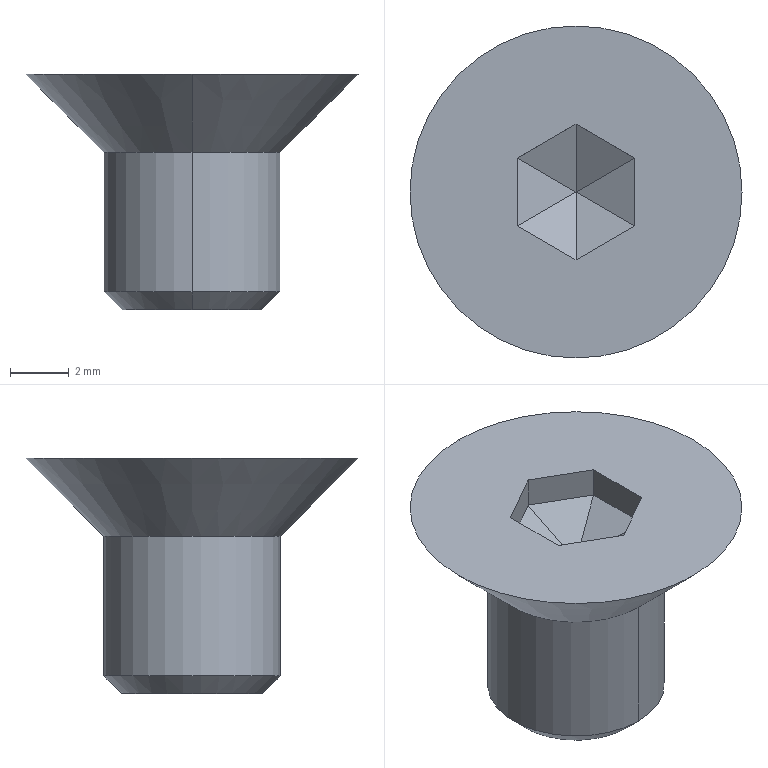Component | SolidWorks | SocketCountersunkHeadScrewM6x8-1 | 1 solid | 21 faces | box 11.3 x 11.3 x 8 mm | volume 289 mm3 | plane 15 | cone 4 | cylinder 2 | commonest cylinder face diameters 6 x2
build123d program:
from build123d import *
from OCP.BRepFilletAPI import BRepFilletAPI_MakeChamfer

# Parameters (mm, degrees)
SKETCH4_R           = 3
BOSS_EXTRUDE2_DEPTH = 8
CUT_EXTRUDE1_DEPTH  = 2.2
CHAMFER3_SIZE       = 1.153
CHAMFER3_SIZE2      = 1.997
CHAMFER4_SIZE       = 0.6


with BuildPart() as part:
    # Sketch2 → Revolve1 (revolve)
    with BuildSketch(Plane.XY, mode=Mode.PRIVATE) as revolve1_sk:
        Polygon((0, -3.72), (0, 0), (5.65, 0), (1.93, -3.72), align=None)
    revolve(revolve1_sk.sketch.rotate(Axis((0, -3.72, 0), (0, 1, 0)), 90), axis=Axis((0, -3.72, 0), (0, 1, 0)))

    # Sketch4 → Boss-Extrude2 (add)
    with BuildSketch(Plane.XZ):
        with Locations(Location((0, 0, 0), (0, 0, 90))):
            Circle(SKETCH4_R)
    extrude(amount=BOSS_EXTRUDE2_DEPTH)

    # Sketch3 → Cut-Extrude1 (cut)
    with BuildSketch(Plane(origin=(0, 0, 0), x_dir=(1, 0, 0), z_dir=(0, 1, 0))):
        Polygon((2, 1.155), (0, 2.309), (-2, 1.155), (-2, -1.155), (0, -2.309), (2, -1.155), align=None)
    extrude(amount=-CUT_EXTRUDE1_DEPTH, mode=Mode.SUBTRACT)

    # Chamfer3: one chamfer whose edges measure the first distance from different faces: ONE call of the kernel's chamfer builder (chamfer() names one face for all edges)
    chamfer3_edges_1 = [part.edges().sort_by_distance(p)[0] for p in [
        (2, -2.2, 0),
    ]]
    chamfer3_side_1 = [part.faces().sort_by_distance(p)[0] for p in [
        (2, -1.1, 0),
    ]]
    chamfer3_edges_2 = [part.edges().sort_by_distance(p)[0] for p in [
        (1, -2.2, 1.732),
    ]]
    chamfer3_side_2 = [part.faces().sort_by_distance(p)[0] for p in [
        (1, -1.1, 1.732),
    ]]
    chamfer3_edges_3 = [part.edges().sort_by_distance(p)[0] for p in [
        (-1, -2.2, 1.732),
    ]]
    chamfer3_side_3 = [part.faces().sort_by_distance(p)[0] for p in [
        (-1, -1.1, 1.732),
    ]]
    chamfer3_edges_4 = [part.edges().sort_by_distance(p)[0] for p in [
        (-2, -2.2, 0),
    ]]
    chamfer3_side_4 = [part.faces().sort_by_distance(p)[0] for p in [
        (-2, -1.1, 0),
    ]]
    chamfer3_edges_5 = [part.edges().sort_by_distance(p)[0] for p in [
        (-1, -2.2, -1.732),
    ]]
    chamfer3_side_5 = [part.faces().sort_by_distance(p)[0] for p in [
        (-1, -1.1, -1.732),
    ]]
    chamfer3_edges_6 = [part.edges().sort_by_distance(p)[0] for p in [
        (1, -2.2, -1.732),
    ]]
    chamfer3_side_6 = [part.faces().sort_by_distance(p)[0] for p in [
        (1, -1.1, -1.732),
    ]]
    chamfer3 = BRepFilletAPI_MakeChamfer(part.part.solid().wrapped)
    for e in chamfer3_edges_1:
        chamfer3.Add(CHAMFER3_SIZE, CHAMFER3_SIZE2, e.wrapped, chamfer3_side_1[0].wrapped)  # the first distance lies on this face
    for e in chamfer3_edges_2:
        chamfer3.Add(CHAMFER3_SIZE, CHAMFER3_SIZE2, e.wrapped, chamfer3_side_2[0].wrapped)  # the first distance lies on this face
    for e in chamfer3_edges_3:
        chamfer3.Add(CHAMFER3_SIZE, CHAMFER3_SIZE2, e.wrapped, chamfer3_side_3[0].wrapped)  # the first distance lies on this face
    for e in chamfer3_edges_4:
        chamfer3.Add(CHAMFER3_SIZE, CHAMFER3_SIZE2, e.wrapped, chamfer3_side_4[0].wrapped)  # the first distance lies on this face
    for e in chamfer3_edges_5:
        chamfer3.Add(CHAMFER3_SIZE, CHAMFER3_SIZE2, e.wrapped, chamfer3_side_5[0].wrapped)  # the first distance lies on this face
    for e in chamfer3_edges_6:
        chamfer3.Add(CHAMFER3_SIZE, CHAMFER3_SIZE2, e.wrapped, chamfer3_side_6[0].wrapped)  # the first distance lies on this face
    add(Compound.cast(chamfer3.Shape()), mode=Mode.REPLACE)

    # Chamfer4
    chamfer4_edges = [part.edges().sort_by_distance(p)[0] for p in [
        (0, -8, -3),
    ]]
    chamfer(chamfer4_edges, length=CHAMFER4_SIZE)


solid = part.part

# Placed as in the assembly
solid = solid.moved(Location((-174.718, -10, 15), (90, 0, 0)))
STEP:
#1=COLOUR_RGB('',0.7922,0.8196,0.9333);
#2=FILL_AREA_STYLE_COLOUR('',#1);
#3=FILL_AREA_STYLE('',(#2));
#4=SURFACE_STYLE_FILL_AREA(#3);
#5=SURFACE_SIDE_STYLE('',(#4));
#6=SURFACE_STYLE_USAGE(.BOTH.,#5);
#7=PRESENTATION_STYLE_ASSIGNMENT((#6));
#8=CARTESIAN_POINT('',(-6.879,-0.2992,0.2756));
#9=VERTEX_POINT('',#8);
#10=CARTESIAN_POINT('',(-6.879,-0.4882,0.2756));
#11=VERTEX_POINT('',#10);
#12=CARTESIAN_POINT('',(-6.879,-0.3937,0.2756));
#13=DIRECTION('',(0.,0.,-1.));
#14=DIRECTION('',(0.,1.,0.));
#15=AXIS2_PLACEMENT_3D('',#12,#13,#14);
#16=CIRCLE('',#15,0.09449);
#17=EDGE_CURVE('',#9,#11,#16,.T.);
#18=ORIENTED_EDGE('',*,*,#17,.F.);
#19=CARTESIAN_POINT('',(-6.879,-0.2756,0.2992));
#20=VERTEX_POINT('',#19);
#21=CARTESIAN_POINT('',(-6.879,-0.2992,0.2756));
#22=DIRECTION('',(0.,0.7071,0.7071));
#23=VECTOR('',#22,39.37);
#24=LINE('',#21,#23);
#25=EDGE_CURVE('',#9,#20,#24,.T.);
#26=ORIENTED_EDGE('',*,*,#25,.T.);
#27=CARTESIAN_POINT('',(-6.879,-0.5118,0.2992));
#28=VERTEX_POINT('',#27);
#29=CARTESIAN_POINT('',(-6.879,-0.3937,0.2992));
#30=DIRECTION('',(0.,-0.,1.));
#31=DIRECTION('',(0.,1.,0.));
#32=AXIS2_PLACEMENT_3D('',#29,#30,#31);
#33=CIRCLE('',#32,0.1181);
#34=EDGE_CURVE('',#28,#20,#33,.T.);
#35=ORIENTED_EDGE('',*,*,#34,.F.);
#36=CARTESIAN_POINT('',(-6.879,-0.4882,0.2756));
#37=DIRECTION('',(0.,-0.7071,0.7071));
#38=VECTOR('',#37,39.37);
#39=LINE('',#36,#38);
#40=EDGE_CURVE('',#11,#28,#39,.T.);
#41=ORIENTED_EDGE('',*,*,#40,.F.);
#42=EDGE_LOOP('',(#18,#26,#35,#41));
#43=FACE_OUTER_BOUND('',#42,.T.);
#44=CARTESIAN_POINT('',(-6.879,-0.3937,0.2756));
#45=DIRECTION('',(0.,-0.,1.));
#46=DIRECTION('',(0.,-1.,-0.));
#47=AXIS2_PLACEMENT_3D('',#44,#45,#46);
#48=CONICAL_SURFACE('',#47,0.09449,0.7854);
#49=ADVANCED_FACE('',(#43),#48,.T.);
#50=ORIENTED_EDGE('',*,*,#34,.T.);
#51=CARTESIAN_POINT('',(-6.879,-0.2756,0.4862));
#52=VERTEX_POINT('',#51);
#53=CARTESIAN_POINT('',(-6.879,-0.2756,0.2756));
#54=DIRECTION('',(0.,-0.,1.));
#55=VECTOR('',#54,39.37);
#56=LINE('',#53,#55);
#57=EDGE_CURVE('',#20,#52,#56,.T.);
#58=ORIENTED_EDGE('',*,*,#57,.T.);
#59=CARTESIAN_POINT('',(-6.879,-0.5118,0.4862));
#60=VERTEX_POINT('',#59);
#61=CARTESIAN_POINT('',(-6.879,-0.3937,0.4862));
#62=DIRECTION('',(0.,-0.,1.));
#63=DIRECTION('',(0.,-1.,-0.));
#64=AXIS2_PLACEMENT_3D('',#61,#62,#63);
#65=CIRCLE('',#64,0.1181);
#66=EDGE_CURVE('',#60,#52,#65,.T.);
#67=ORIENTED_EDGE('',*,*,#66,.F.);
#68=CARTESIAN_POINT('',(-6.879,-0.5118,0.2756));
#69=DIRECTION('',(0.,-0.,1.));
#70=VECTOR('',#69,39.37);
#71=LINE('',#68,#70);
#72=EDGE_CURVE('',#28,#60,#71,.T.);
#73=ORIENTED_EDGE('',*,*,#72,.F.);
#74=EDGE_LOOP('',(#50,#58,#67,#73));
#75=FACE_OUTER_BOUND('',#74,.T.);
#76=CARTESIAN_POINT('',(-6.879,-0.3937,0.2756));
#77=DIRECTION('',(0.,-0.,1.));
#78=DIRECTION('',(0.,-1.,-0.));
#79=AXIS2_PLACEMENT_3D('',#76,#77,#78);
#80=CYLINDRICAL_SURFACE('',#79,0.1181);
#81=ADVANCED_FACE('',(#75),#80,.T.);
#82=ORIENTED_EDGE('',*,*,#66,.T.);
#83=CARTESIAN_POINT('',(-6.879,-0.1713,0.5906));
#84=VERTEX_POINT('',#83);
#85=CARTESIAN_POINT('',(-6.879,-0.3177,0.4441));
#86=DIRECTION('',(0.,0.7071,0.7071));
#87=VECTOR('',#86,39.37);
#88=LINE('',#85,#87);
#89=EDGE_CURVE('',#52,#84,#88,.T.);
#90=ORIENTED_EDGE('',*,*,#89,.T.);
#91=CARTESIAN_POINT('',(-6.879,-0.6161,0.5906));
#92=VERTEX_POINT('',#91);
#93=CARTESIAN_POINT('',(-6.879,-0.3937,0.5906));
#94=DIRECTION('',(0.,0.,-1.));
#95=DIRECTION('',(0.,1.,0.));
#96=AXIS2_PLACEMENT_3D('',#93,#94,#95);
#97=CIRCLE('',#96,0.2224);
#98=EDGE_CURVE('',#84,#92,#97,.T.);
#99=ORIENTED_EDGE('',*,*,#98,.T.);
#100=CARTESIAN_POINT('',(-6.879,-0.4697,0.4441));
#101=DIRECTION('',(0.,-0.7071,0.7071));
#102=VECTOR('',#101,39.37);
#103=LINE('',#100,#102);
#104=EDGE_CURVE('',#60,#92,#103,.T.);
#105=ORIENTED_EDGE('',*,*,#104,.F.);
#106=EDGE_LOOP('',(#82,#90,#99,#105));
#107=FACE_OUTER_BOUND('',#106,.T.);
#108=CARTESIAN_POINT('',(-6.879,-0.3937,0.4441));
#109=DIRECTION('',(0.,-0.,1.));
#110=DIRECTION('',(0.,-1.,-0.));
#111=AXIS2_PLACEMENT_3D('',#108,#109,#110);
#112=CONICAL_SURFACE('',#111,0.07598,0.7854);
#113=ADVANCED_FACE('',(#107),#112,.T.);
#114=ORIENTED_EDGE('',*,*,#89,.F.);
#115=CARTESIAN_POINT('',(-6.879,-0.3937,0.4862));
#116=DIRECTION('',(0.,-0.,1.));
#117=DIRECTION('',(0.,-1.,-0.));
#118=AXIS2_PLACEMENT_3D('',#115,#116,#117);
#119=CIRCLE('',#118,0.1181);
#120=EDGE_CURVE('',#52,#60,#119,.T.);
#121=ORIENTED_EDGE('',*,*,#120,.T.);
#122=ORIENTED_EDGE('',*,*,#104,.T.);
#123=CARTESIAN_POINT('',(-6.879,-0.3937,0.5906));
#124=DIRECTION('',(0.,0.,-1.));
#125=DIRECTION('',(0.,1.,0.));
#126=AXIS2_PLACEMENT_3D('',#123,#124,#125);
#127=CIRCLE('',#126,0.2224);
#128=EDGE_CURVE('',#92,#84,#127,.T.);
#129=ORIENTED_EDGE('',*,*,#128,.T.);
#130=EDGE_LOOP('',(#114,#121,#122,#129));
#131=FACE_OUTER_BOUND('',#130,.T.);
#132=CARTESIAN_POINT('',(-6.879,-0.3937,0.4441));
#133=DIRECTION('',(0.,-0.,1.));
#134=DIRECTION('',(0.,-1.,-0.));
#135=AXIS2_PLACEMENT_3D('',#132,#133,#134);
#136=CONICAL_SURFACE('',#135,0.07598,0.7854);
#137=ADVANCED_FACE('',(#131),#136,.T.);
#138=CARTESIAN_POINT('',(-6.8,-0.4392,0.5906));
#139=VERTEX_POINT('',#138);
#140=CARTESIAN_POINT('',(-6.8,-0.3482,0.5906));
#141=VERTEX_POINT('',#140);
#142=CARTESIAN_POINT('',(-6.8,-0.4392,0.5906));
#143=DIRECTION('',(-0.,1.,0.));
#144=VECTOR('',#143,39.37);
#145=LINE('',#142,#144);
#146=EDGE_CURVE('',#139,#141,#145,.T.);
#147=ORIENTED_EDGE('',*,*,#146,.F.);
#148=CARTESIAN_POINT('',(-6.879,-0.4846,0.5906));
#149=VERTEX_POINT('',#148);
#150=CARTESIAN_POINT('',(-6.879,-0.4846,0.5906));
#151=DIRECTION('',(0.866,0.5,0.));
#152=VECTOR('',#151,39.37);
#153=LINE('',#150,#152);
#154=EDGE_CURVE('',#149,#139,#153,.T.);
#155=ORIENTED_EDGE('',*,*,#154,.F.);
#156=CARTESIAN_POINT('',(-6.957,-0.4392,0.5906));
#157=VERTEX_POINT('',#156);
#158=CARTESIAN_POINT('',(-6.957,-0.4392,0.5906));
#159=DIRECTION('',(0.866,-0.5,-0.));
#160=VECTOR('',#159,39.37);
#161=LINE('',#158,#160);
#162=EDGE_CURVE('',#157,#149,#161,.T.);
#163=ORIENTED_EDGE('',*,*,#162,.F.);
#164=CARTESIAN_POINT('',(-6.957,-0.3482,0.5906));
#165=VERTEX_POINT('',#164);
#166=CARTESIAN_POINT('',(-6.957,-0.3482,0.5906));
#167=DIRECTION('',(0.,-1.,-0.));
#168=VECTOR('',#167,39.37);
#169=LINE('',#166,#168);
#170=EDGE_CURVE('',#165,#157,#169,.T.);
#171=ORIENTED_EDGE('',*,*,#170,.F.);
#172=CARTESIAN_POINT('',(-6.879,-0.3028,0.5906));
#173=VERTEX_POINT('',#172);
#174=CARTESIAN_POINT('',(-6.879,-0.3028,0.5906));
#175=DIRECTION('',(-0.866,-0.5,-0.));
#176=VECTOR('',#175,39.37);
#177=LINE('',#174,#176);
#178=EDGE_CURVE('',#173,#165,#177,.T.);
#179=ORIENTED_EDGE('',*,*,#178,.F.);
#180=CARTESIAN_POINT('',(-6.8,-0.3482,0.5906));
#181=DIRECTION('',(-0.866,0.5,0.));
#182=VECTOR('',#181,39.37);
#183=LINE('',#180,#182);
#184=EDGE_CURVE('',#141,#173,#183,.T.);
#185=ORIENTED_EDGE('',*,*,#184,.F.);
#186=EDGE_LOOP('',(#147,#155,#163,#171,#179,#185));
#187=FACE_BOUND('',#186,.T.);
#188=ORIENTED_EDGE('',*,*,#128,.F.);
#189=ORIENTED_EDGE('',*,*,#98,.F.);
#190=EDGE_LOOP('',(#188,#189));
#191=FACE_OUTER_BOUND('',#190,.T.);
#192=CARTESIAN_POINT('',(-6.879,-0.3937,0.5906));
#193=DIRECTION('',(0.,-0.,1.));
#194=DIRECTION('',(0.,-1.,-0.));
#195=AXIS2_PLACEMENT_3D('',#192,#193,#194);
#196=PLANE('',#195);
#197=ADVANCED_FACE('',(#187,#191),#196,.T.);
#198=ORIENTED_EDGE('',*,*,#57,.F.);
#199=CARTESIAN_POINT('',(-6.879,-0.3937,0.2992));
#200=DIRECTION('',(0.,-0.,1.));
#201=DIRECTION('',(0.,1.,0.));
#202=AXIS2_PLACEMENT_3D('',#199,#200,#201);
#203=CIRCLE('',#202,0.1181);
#204=EDGE_CURVE('',#20,#28,#203,.T.);
#205=ORIENTED_EDGE('',*,*,#204,.T.);
#206=ORIENTED_EDGE('',*,*,#72,.T.);
#207=ORIENTED_EDGE('',*,*,#120,.F.);
#208=EDGE_LOOP('',(#198,#205,#206,#207));
#209=FACE_OUTER_BOUND('',#208,.T.);
#210=CARTESIAN_POINT('',(-6.879,-0.3937,0.2756));
#211=DIRECTION('',(0.,-0.,1.));
#212=DIRECTION('',(0.,-1.,-0.));
#213=AXIS2_PLACEMENT_3D('',#210,#211,#212);
#214=CYLINDRICAL_SURFACE('',#213,0.1181);
#215=ADVANCED_FACE('',(#209),#214,.T.);
#216=CARTESIAN_POINT('',(-6.879,-0.3937,0.2756));
#217=DIRECTION('',(0.,0.,-1.));
#218=DIRECTION('',(0.,1.,0.));
#219=AXIS2_PLACEMENT_3D('',#216,#217,#218);
#220=CIRCLE('',#219,0.09449);
#221=EDGE_CURVE('',#11,#9,#220,.T.);
#222=ORIENTED_EDGE('',*,*,#221,.T.);
#223=ORIENTED_EDGE('',*,*,#17,.T.);
#224=EDGE_LOOP('',(#222,#223));
#225=FACE_OUTER_BOUND('',#224,.T.);
#226=CARTESIAN_POINT('',(-6.879,-0.3937,0.2756));
#227=DIRECTION('',(0.,0.,-1.));
#228=DIRECTION('',(0.,1.,0.));
#229=AXIS2_PLACEMENT_3D('',#226,#227,#228);
#230=PLANE('',#229);
#231=ADVANCED_FACE('',(#225),#230,.T.);
#232=CARTESIAN_POINT('',(-6.8,-0.3482,0.5493));
#233=VERTEX_POINT('',#232);
#234=CARTESIAN_POINT('',(-6.8,-0.3482,0.5039));
#235=DIRECTION('',(0.,-0.,1.));
#236=VECTOR('',#235,39.37);
#237=LINE('',#234,#236);
#238=EDGE_CURVE('',#233,#141,#237,.T.);
#239=ORIENTED_EDGE('',*,*,#238,.F.);
#240=CARTESIAN_POINT('',(-6.8,-0.4392,0.5493));
#241=VERTEX_POINT('',#240);
#242=CARTESIAN_POINT('',(-6.8,-0.4392,0.5493));
#243=DIRECTION('',(0.,-1.,-0.));
#244=VECTOR('',#243,39.37);
#245=LINE('',#242,#244);
#246=EDGE_CURVE('',#233,#241,#245,.T.);
#247=ORIENTED_EDGE('',*,*,#246,.T.);
#248=CARTESIAN_POINT('',(-6.8,-0.4392,0.5039));
#249=DIRECTION('',(0.,-0.,1.));
#250=VECTOR('',#249,39.37);
#251=LINE('',#248,#250);
#252=EDGE_CURVE('',#241,#139,#251,.T.);
#253=ORIENTED_EDGE('',*,*,#252,.T.);
#254=ORIENTED_EDGE('',*,*,#146,.T.);
#255=EDGE_LOOP('',(#239,#247,#253,#254));
#256=FACE_OUTER_BOUND('',#255,.T.);
#257=CARTESIAN_POINT('',(-6.8,-0.4392,0.5039));
#258=DIRECTION('',(1.,0.,0.));
#259=DIRECTION('',(-0.,1.,0.));
#260=AXIS2_PLACEMENT_3D('',#257,#258,#259);
#261=PLANE('',#260);
#262=ADVANCED_FACE('',(#256),#261,.F.);
#263=ORIENTED_EDGE('',*,*,#252,.F.);
#264=CARTESIAN_POINT('',(-6.879,-0.4846,0.5493));
#265=VERTEX_POINT('',#264);
#266=CARTESIAN_POINT('',(-6.879,-0.4846,0.5493));
#267=DIRECTION('',(-0.866,-0.5,-0.));
#268=VECTOR('',#267,39.37);
#269=LINE('',#266,#268);
#270=EDGE_CURVE('',#241,#265,#269,.T.);
#271=ORIENTED_EDGE('',*,*,#270,.T.);
#272=CARTESIAN_POINT('',(-6.879,-0.4846,0.5039));
#273=DIRECTION('',(0.,-0.,1.));
#274=VECTOR('',#273,39.37);
#275=LINE('',#272,#274);
#276=EDGE_CURVE('',#265,#149,#275,.T.);
#277=ORIENTED_EDGE('',*,*,#276,.T.);
#278=ORIENTED_EDGE('',*,*,#154,.T.);
#279=EDGE_LOOP('',(#263,#271,#277,#278));
#280=FACE_OUTER_BOUND('',#279,.T.);
#281=CARTESIAN_POINT('',(-6.879,-0.4846,0.5039));
#282=DIRECTION('',(0.5,-0.866,-0.));
#283=DIRECTION('',(0.866,0.5,0.));
#284=AXIS2_PLACEMENT_3D('',#281,#282,#283);
#285=PLANE('',#284);
#286=ADVANCED_FACE('',(#280),#285,.F.);
#287=ORIENTED_EDGE('',*,*,#276,.F.);
#288=CARTESIAN_POINT('',(-6.957,-0.4392,0.5493));
#289=VERTEX_POINT('',#288);
#290=CARTESIAN_POINT('',(-6.957,-0.4392,0.5493));
#291=DIRECTION('',(-0.866,0.5,0.));
#292=VECTOR('',#291,39.37);
#293=LINE('',#290,#292);
#294=EDGE_CURVE('',#265,#289,#293,.T.);
#295=ORIENTED_EDGE('',*,*,#294,.T.);
#296=CARTESIAN_POINT('',(-6.957,-0.4392,0.5039));
#297=DIRECTION('',(0.,-0.,1.));
#298=VECTOR('',#297,39.37);
#299=LINE('',#296,#298);
#300=EDGE_CURVE('',#289,#157,#299,.T.);
#301=ORIENTED_EDGE('',*,*,#300,.T.);
#302=ORIENTED_EDGE('',*,*,#162,.T.);
#303=EDGE_LOOP('',(#287,#295,#301,#302));
#304=FACE_OUTER_BOUND('',#303,.T.);
#305=CARTESIAN_POINT('',(-6.957,-0.4392,0.5039));
#306=DIRECTION('',(-0.5,-0.866,-0.));
#307=DIRECTION('',(0.866,-0.5,-0.));
#308=AXIS2_PLACEMENT_3D('',#305,#306,#307);
#309=PLANE('',#308);
#310=ADVANCED_FACE('',(#304),#309,.F.);
#311=ORIENTED_EDGE('',*,*,#300,.F.);
#312=CARTESIAN_POINT('',(-6.957,-0.3482,0.5493));
#313=VERTEX_POINT('',#312);
#314=CARTESIAN_POINT('',(-6.957,-0.3482,0.5493));
#315=DIRECTION('',(0.,1.,0.));
#316=VECTOR('',#315,39.37);
#317=LINE('',#314,#316);
#318=EDGE_CURVE('',#289,#313,#317,.T.);
#319=ORIENTED_EDGE('',*,*,#318,.T.);
#320=CARTESIAN_POINT('',(-6.957,-0.3482,0.5039));
#321=DIRECTION('',(0.,-0.,1.));
#322=VECTOR('',#321,39.37);
#323=LINE('',#320,#322);
#324=EDGE_CURVE('',#313,#165,#323,.T.);
#325=ORIENTED_EDGE('',*,*,#324,.T.);
#326=ORIENTED_EDGE('',*,*,#170,.T.);
#327=EDGE_LOOP('',(#311,#319,#325,#326));
#328=FACE_OUTER_BOUND('',#327,.T.);
#329=CARTESIAN_POINT('',(-6.957,-0.3482,0.5039));
#330=DIRECTION('',(-1.,0.,0.));
#331=DIRECTION('',(0.,-1.,-0.));
#332=AXIS2_PLACEMENT_3D('',#329,#330,#331);
#333=PLANE('',#332);
#334=ADVANCED_FACE('',(#328),#333,.F.);
#335=ORIENTED_EDGE('',*,*,#324,.F.);
#336=CARTESIAN_POINT('',(-6.879,-0.3028,0.5493));
#337=VERTEX_POINT('',#336);
#338=CARTESIAN_POINT('',(-6.879,-0.3028,0.5493));
#339=DIRECTION('',(0.866,0.5,0.));
#340=VECTOR('',#339,39.37);
#341=LINE('',#338,#340);
#342=EDGE_CURVE('',#313,#337,#341,.T.);
#343=ORIENTED_EDGE('',*,*,#342,.T.);
#344=CARTESIAN_POINT('',(-6.879,-0.3028,0.5039));
#345=DIRECTION('',(0.,-0.,1.));
#346=VECTOR('',#345,39.37);
#347=LINE('',#344,#346);
#348=EDGE_CURVE('',#337,#173,#347,.T.);
#349=ORIENTED_EDGE('',*,*,#348,.T.);
#350=ORIENTED_EDGE('',*,*,#178,.T.);
#351=EDGE_LOOP('',(#335,#343,#349,#350));
#352=FACE_OUTER_BOUND('',#351,.T.);
#353=CARTESIAN_POINT('',(-6.879,-0.3028,0.5039));
#354=DIRECTION('',(-0.5,0.866,0.));
#355=DIRECTION('',(-0.866,-0.5,-0.));
#356=AXIS2_PLACEMENT_3D('',#353,#354,#355);
#357=PLANE('',#356);
#358=ADVANCED_FACE('',(#352),#357,.F.);
#359=ORIENTED_EDGE('',*,*,#348,.F.);
#360=CARTESIAN_POINT('',(-6.8,-0.3482,0.5493));
#361=DIRECTION('',(0.866,-0.5,-0.));
#362=VECTOR('',#361,39.37);
#363=LINE('',#360,#362);
#364=EDGE_CURVE('',#337,#233,#363,.T.);
#365=ORIENTED_EDGE('',*,*,#364,.T.);
#366=ORIENTED_EDGE('',*,*,#238,.T.);
#367=ORIENTED_EDGE('',*,*,#184,.T.);
#368=EDGE_LOOP('',(#359,#365,#366,#367));
#369=FACE_OUTER_BOUND('',#368,.T.);
#370=CARTESIAN_POINT('',(-6.8,-0.3482,0.5039));
#371=DIRECTION('',(0.5,0.866,0.));
#372=DIRECTION('',(-0.866,0.5,0.));
#373=AXIS2_PLACEMENT_3D('',#370,#371,#372);
#374=PLANE('',#373);
#375=ADVANCED_FACE('',(#369),#374,.F.);
#376=CARTESIAN_POINT('',(-6.879,-0.3936,0.5039));
#377=VERTEX_POINT('',#376);
#378=CARTESIAN_POINT('',(-6.879,-0.3938,0.5039));
#379=VERTEX_POINT('',#378);
#380=CARTESIAN_POINT('',(-6.879,-0.3937,0.5039));
#381=DIRECTION('',(0.,-1.,-0.));
#382=VECTOR('',#381,39.37);
#383=LINE('',#380,#382);
#384=EDGE_CURVE('',#377,#379,#383,.T.);
#385=ORIENTED_EDGE('',*,*,#384,.T.);
#386=CARTESIAN_POINT('',(-6.879,-0.3939,0.5039));
#387=VERTEX_POINT('',#386);
#388=CARTESIAN_POINT('',(-6.879,-0.3938,0.5039));
#389=DIRECTION('',(0.866,-0.5,-0.));
#390=VECTOR('',#389,39.37);
#391=LINE('',#388,#390);
#392=EDGE_CURVE('',#379,#387,#391,.T.);
#393=ORIENTED_EDGE('',*,*,#392,.T.);
#394=CARTESIAN_POINT('',(-6.879,-0.3938,0.5039));
#395=VERTEX_POINT('',#394);
#396=CARTESIAN_POINT('',(-6.879,-0.3938,0.5039));
#397=DIRECTION('',(0.866,0.5,0.));
#398=VECTOR('',#397,39.37);
#399=LINE('',#396,#398);
#400=EDGE_CURVE('',#387,#395,#399,.T.);
#401=ORIENTED_EDGE('',*,*,#400,.T.);
#402=CARTESIAN_POINT('',(-6.879,-0.3936,0.5039));
#403=VERTEX_POINT('',#402);
#404=CARTESIAN_POINT('',(-6.879,-0.3937,0.5039));
#405=DIRECTION('',(-0.,1.,0.));
#406=VECTOR('',#405,39.37);
#407=LINE('',#404,#406);
#408=EDGE_CURVE('',#395,#403,#407,.T.);
#409=ORIENTED_EDGE('',*,*,#408,.T.);
#410=CARTESIAN_POINT('',(-6.879,-0.3935,0.5039));
#411=VERTEX_POINT('',#410);
#412=CARTESIAN_POINT('',(-6.879,-0.3936,0.5039));
#413=DIRECTION('',(-0.866,0.5,0.));
#414=VECTOR('',#413,39.37);
#415=LINE('',#412,#414);
#416=EDGE_CURVE('',#403,#411,#415,.T.);
#417=ORIENTED_EDGE('',*,*,#416,.T.);
#418=CARTESIAN_POINT('',(-6.879,-0.3936,0.5039));
#419=DIRECTION('',(-0.866,-0.5,-0.));
#420=VECTOR('',#419,39.37);
#421=LINE('',#418,#420);
#422=EDGE_CURVE('',#411,#377,#421,.T.);
#423=ORIENTED_EDGE('',*,*,#422,.T.);
#424=EDGE_LOOP('',(#385,#393,#401,#409,#417,#423));
#425=FACE_OUTER_BOUND('',#424,.T.);
#426=CARTESIAN_POINT('',(-6.879,-0.3937,0.5039));
#427=DIRECTION('',(0.,-0.,1.));
#428=DIRECTION('',(0.,-1.,-0.));
#429=AXIS2_PLACEMENT_3D('',#426,#427,#428);
#430=PLANE('',#429);
#431=ADVANCED_FACE('',(#425),#430,.T.);
#432=CARTESIAN_POINT('',(-6.879,-0.3936,0.5039));
#433=DIRECTION('',(-0.7746,-0.4472,-0.4472));
#434=VECTOR('',#433,39.37);
#435=LINE('',#432,#434);
#436=EDGE_CURVE('',#233,#403,#435,.T.);
#437=ORIENTED_EDGE('',*,*,#436,.F.);
#438=ORIENTED_EDGE('',*,*,#364,.F.);
#439=CARTESIAN_POINT('',(-6.879,-0.3936,0.5039));
#440=DIRECTION('',(0.,0.8944,0.4472));
#441=VECTOR('',#440,39.37);
#442=LINE('',#439,#441);
#443=EDGE_CURVE('',#411,#337,#442,.T.);
#444=ORIENTED_EDGE('',*,*,#443,.F.);
#445=ORIENTED_EDGE('',*,*,#416,.F.);
#446=EDGE_LOOP('',(#437,#438,#444,#445));
#447=FACE_OUTER_BOUND('',#446,.T.);
#448=CARTESIAN_POINT('',(-6.879,-0.3936,0.5039));
#449=DIRECTION('',(0.25,0.433,-0.866));
#450=DIRECTION('',(-0.866,0.5,0.));
#451=AXIS2_PLACEMENT_3D('',#448,#449,#450);
#452=PLANE('',#451);
#453=ADVANCED_FACE('',(#447),#452,.F.);
#454=ORIENTED_EDGE('',*,*,#443,.T.);
#455=ORIENTED_EDGE('',*,*,#342,.F.);
#456=CARTESIAN_POINT('',(-6.879,-0.3936,0.5039));
#457=DIRECTION('',(-0.7746,0.4472,0.4472));
#458=VECTOR('',#457,39.37);
#459=LINE('',#456,#458);
#460=EDGE_CURVE('',#377,#313,#459,.T.);
#461=ORIENTED_EDGE('',*,*,#460,.F.);
#462=ORIENTED_EDGE('',*,*,#422,.F.);
#463=EDGE_LOOP('',(#454,#455,#461,#462));
#464=FACE_OUTER_BOUND('',#463,.T.);
#465=CARTESIAN_POINT('',(-6.879,-0.3936,0.5039));
#466=DIRECTION('',(-0.25,0.433,-0.866));
#467=DIRECTION('',(-0.866,-0.5,-0.));
#468=AXIS2_PLACEMENT_3D('',#465,#466,#467);
#469=PLANE('',#468);
#470=ADVANCED_FACE('',(#464),#469,.F.);
#471=ORIENTED_EDGE('',*,*,#436,.T.);
#472=ORIENTED_EDGE('',*,*,#408,.F.);
#473=CARTESIAN_POINT('',(-6.879,-0.3938,0.5039));
#474=DIRECTION('',(-0.7746,0.4472,-0.4472));
#475=VECTOR('',#474,39.37);
#476=LINE('',#473,#475);
#477=EDGE_CURVE('',#241,#395,#476,.T.);
#478=ORIENTED_EDGE('',*,*,#477,.F.);
#479=ORIENTED_EDGE('',*,*,#246,.F.);
#480=EDGE_LOOP('',(#471,#472,#478,#479));
#481=FACE_OUTER_BOUND('',#480,.T.);
#482=CARTESIAN_POINT('',(-6.879,-0.3937,0.5039));
#483=DIRECTION('',(0.5,0.,-0.866));
#484=DIRECTION('',(-0.,1.,0.));
#485=AXIS2_PLACEMENT_3D('',#482,#483,#484);
#486=PLANE('',#485);
#487=ADVANCED_FACE('',(#481),#486,.F.);
#488=ORIENTED_EDGE('',*,*,#460,.T.);
#489=ORIENTED_EDGE('',*,*,#318,.F.);
#490=CARTESIAN_POINT('',(-6.879,-0.3938,0.5039));
#491=DIRECTION('',(-0.7746,-0.4472,0.4472));
#492=VECTOR('',#491,39.37);
#493=LINE('',#490,#492);
#494=EDGE_CURVE('',#379,#289,#493,.T.);
#495=ORIENTED_EDGE('',*,*,#494,.F.);
#496=ORIENTED_EDGE('',*,*,#384,.F.);
#497=EDGE_LOOP('',(#488,#489,#495,#496));
#498=FACE_OUTER_BOUND('',#497,.T.);
#499=CARTESIAN_POINT('',(-6.879,-0.3937,0.5039));
#500=DIRECTION('',(-0.5,0.,-0.866));
#501=DIRECTION('',(0.,-1.,-0.));
#502=AXIS2_PLACEMENT_3D('',#499,#500,#501);
#503=PLANE('',#502);
#504=ADVANCED_FACE('',(#498),#503,.F.);
#505=ORIENTED_EDGE('',*,*,#477,.T.);
#506=ORIENTED_EDGE('',*,*,#400,.F.);
#507=CARTESIAN_POINT('',(-6.879,-0.3938,0.5039));
#508=DIRECTION('',(0.,0.8944,-0.4472));
#509=VECTOR('',#508,39.37);
#510=LINE('',#507,#509);
#511=EDGE_CURVE('',#265,#387,#510,.T.);
#512=ORIENTED_EDGE('',*,*,#511,.F.);
#513=ORIENTED_EDGE('',*,*,#270,.F.);
#514=EDGE_LOOP('',(#505,#506,#512,#513));
#515=FACE_OUTER_BOUND('',#514,.T.);
#516=CARTESIAN_POINT('',(-6.879,-0.3938,0.5039));
#517=DIRECTION('',(0.25,-0.433,-0.866));
#518=DIRECTION('',(0.866,0.5,0.));
#519=AXIS2_PLACEMENT_3D('',#516,#517,#518);
#520=PLANE('',#519);
#521=ADVANCED_FACE('',(#515),#520,.F.);
#522=ORIENTED_EDGE('',*,*,#494,.T.);
#523=ORIENTED_EDGE('',*,*,#294,.F.);
#524=ORIENTED_EDGE('',*,*,#511,.T.);
#525=ORIENTED_EDGE('',*,*,#392,.F.);
#526=EDGE_LOOP('',(#522,#523,#524,#525));
#527=FACE_OUTER_BOUND('',#526,.T.);
#528=CARTESIAN_POINT('',(-6.879,-0.3938,0.5039));
#529=DIRECTION('',(-0.25,-0.433,-0.866));
#530=DIRECTION('',(0.866,-0.5,-0.));
#531=AXIS2_PLACEMENT_3D('',#528,#529,#530);
#532=PLANE('',#531);
#533=ADVANCED_FACE('',(#527),#532,.F.);
#534=ORIENTED_EDGE('',*,*,#25,.F.);
#535=ORIENTED_EDGE('',*,*,#221,.F.);
#536=ORIENTED_EDGE('',*,*,#40,.T.);
#537=ORIENTED_EDGE('',*,*,#204,.F.);
#538=EDGE_LOOP('',(#534,#535,#536,#537));
#539=FACE_OUTER_BOUND('',#538,.T.);
#540=CARTESIAN_POINT('',(-6.879,-0.3937,0.2756));
#541=DIRECTION('',(0.,-0.,1.));
#542=DIRECTION('',(0.,-1.,-0.));
#543=AXIS2_PLACEMENT_3D('',#540,#541,#542);
#544=CONICAL_SURFACE('',#543,0.09449,0.7854);
#545=ADVANCED_FACE('',(#539),#544,.T.);
#546=CLOSED_SHELL('',(#49,#81,#113,#137,#197,#215,#231,#262,#286,#310,#334,#358,#375,#431,#453,#470,#487,#504,#521,#533,#545));
#547=MANIFOLD_SOLID_BREP('',#546);
#548=STYLED_ITEM('',(#7),#547);
#549=PRESENTATION_LAYER_ASSIGNMENT('','',(#548));
#550=CARTESIAN_POINT('',(0.,0.,0.));
#551=DIRECTION('',(0.,0.,1.));
#552=DIRECTION('',(1.,0.,0.));
#553=AXIS2_PLACEMENT_3D('',#550,#551,#552);
#554=(LENGTH_UNIT()NAMED_UNIT(*)SI_UNIT($,.METRE.));
#555=LENGTH_MEASURE_WITH_UNIT(LENGTH_MEASURE(0.0254),#554);
#556=DIMENSIONAL_EXPONENTS(1.,0.,0.,0.,0.,0.,0.);
#557=(CONVERSION_BASED_UNIT('',#555)LENGTH_UNIT()NAMED_UNIT(#556));
#558=UNCERTAINTY_MEASURE_WITH_UNIT(LENGTH_MEASURE(0.00001),#557,'','');
#559=(NAMED_UNIT(*)PLANE_ANGLE_UNIT()SI_UNIT($,.RADIAN.));
#560=(NAMED_UNIT(*)SI_UNIT($,.STERADIAN.)SOLID_ANGLE_UNIT());
#561=(GEOMETRIC_REPRESENTATION_CONTEXT(3)GLOBAL_UNCERTAINTY_ASSIGNED_CONTEXT((#558))GLOBAL_UNIT_ASSIGNED_CONTEXT((#557,#559,#560))REPRESENTATION_CONTEXT('',''));
#562=ADVANCED_BREP_SHAPE_REPRESENTATION('',(#547,#553),#561);
#563=(LENGTH_UNIT()NAMED_UNIT(*)SI_UNIT($,.METRE.));
#564=LENGTH_MEASURE_WITH_UNIT(LENGTH_MEASURE(0.0254),#563);
#565=DIMENSIONAL_EXPONENTS(1.,0.,0.,0.,0.,0.,0.);
#566=(CONVERSION_BASED_UNIT('',#564)LENGTH_UNIT()NAMED_UNIT(#565));
#567=UNCERTAINTY_MEASURE_WITH_UNIT(LENGTH_MEASURE(0.00001),#566,'','');
#568=(NAMED_UNIT(*)PLANE_ANGLE_UNIT()SI_UNIT($,.RADIAN.));
#569=(NAMED_UNIT(*)SI_UNIT($,.STERADIAN.)SOLID_ANGLE_UNIT());
#570=(GEOMETRIC_REPRESENTATION_CONTEXT(3)GLOBAL_UNCERTAINTY_ASSIGNED_CONTEXT((#567))GLOBAL_UNIT_ASSIGNED_CONTEXT((#566,#568,#569))REPRESENTATION_CONTEXT('',''));
#571=MECHANICAL_DESIGN_GEOMETRIC_PRESENTATION_REPRESENTATION('',(#548),#570);